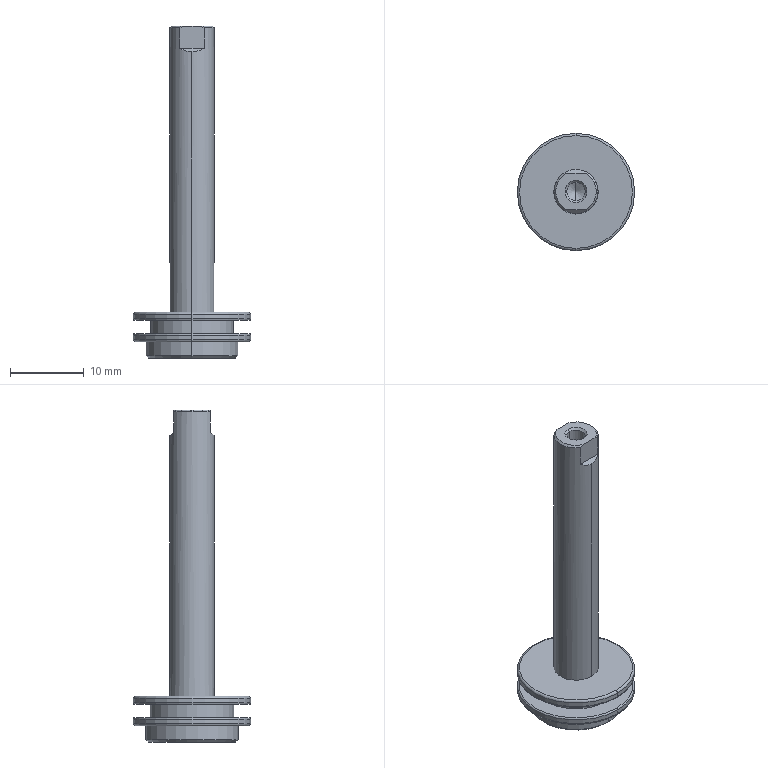Component | SolidWorks | SDA_16x25_0-1_SDA_16x2525_r-1 | 1 solid | 38 faces | box 15.9 x 15.9 x 45 mm | volume 1937 mm3 | cylinder 12 | plane 10 | cone 8 | torus 8 | commonest cylinder face diameters 15.9 x4 2.459 x2 12.5 x2 11.3 x2 6 x2
STEP:
#1=COLOUR_RGB('',0.7922,0.8196,0.9333);
#2=FILL_AREA_STYLE_COLOUR('',#1);
#3=FILL_AREA_STYLE('',(#2));
#4=SURFACE_STYLE_FILL_AREA(#3);
#5=SURFACE_SIDE_STYLE('',(#4));
#6=SURFACE_STYLE_USAGE(.BOTH.,#5);
#7=PRESENTATION_STYLE_ASSIGNMENT((#6));
#8=CARTESIAN_POINT('',(-0.2723,0.7951,0.8728));
#9=VERTEX_POINT('',#8);
#10=CARTESIAN_POINT('',(-0.2723,0.8435,0.9007));
#11=VERTEX_POINT('',#10);
#12=CARTESIAN_POINT('',(-0.2723,0.7951,0.8728));
#13=DIRECTION('',(0.,0.866,0.5));
#14=VECTOR('',#13,39.37);
#15=LINE('',#12,#14);
#16=EDGE_CURVE('',#9,#11,#15,.T.);
#17=ORIENTED_EDGE('',*,*,#16,.F.);
#18=CARTESIAN_POINT('',(-0.2723,0.7467,0.9007));
#19=VERTEX_POINT('',#18);
#20=CARTESIAN_POINT('',(-0.2723,0.7951,0.8728));
#21=DIRECTION('',(-0.,-0.866,0.5));
#22=VECTOR('',#21,39.37);
#23=LINE('',#20,#22);
#24=EDGE_CURVE('',#9,#19,#23,.T.);
#25=ORIENTED_EDGE('',*,*,#24,.T.);
#26=CARTESIAN_POINT('',(-0.2723,0.7951,0.9007));
#27=DIRECTION('',(-0.,0.,1.));
#28=DIRECTION('',(0.,1.,0.));
#29=AXIS2_PLACEMENT_3D('',#26,#27,#28);
#30=CIRCLE('',#29,0.04841);
#31=EDGE_CURVE('',#19,#11,#30,.T.);
#32=ORIENTED_EDGE('',*,*,#31,.T.);
#33=EDGE_LOOP('',(#17,#25,#32));
#34=FACE_OUTER_BOUND('',#33,.T.);
#35=CARTESIAN_POINT('',(-0.2723,0.7951,40.243));
#36=DIRECTION('',(-0.,0.,1.));
#37=DIRECTION('',(0.,1.,0.));
#38=AXIS2_PLACEMENT_3D('',#35,#36,#37);
#39=CONICAL_SURFACE('',#38,68.191,1.047);
#40=ADVANCED_FACE('',(#34),#39,.F.);
#41=ORIENTED_EDGE('',*,*,#31,.F.);
#42=CARTESIAN_POINT('',(-0.2723,0.7467,1.174));
#43=VERTEX_POINT('',#42);
#44=CARTESIAN_POINT('',(-0.2723,0.7467,0.8728));
#45=DIRECTION('',(-0.,0.,1.));
#46=VECTOR('',#45,39.37);
#47=LINE('',#44,#46);
#48=EDGE_CURVE('',#19,#43,#47,.T.);
#49=ORIENTED_EDGE('',*,*,#48,.T.);
#50=CARTESIAN_POINT('',(-0.2723,0.8435,1.174));
#51=VERTEX_POINT('',#50);
#52=CARTESIAN_POINT('',(-0.2723,0.7951,1.174));
#53=DIRECTION('',(-0.,0.,1.));
#54=DIRECTION('',(0.,1.,0.));
#55=AXIS2_PLACEMENT_3D('',#52,#53,#54);
#56=CIRCLE('',#55,0.04841);
#57=EDGE_CURVE('',#43,#51,#56,.T.);
#58=ORIENTED_EDGE('',*,*,#57,.T.);
#59=CARTESIAN_POINT('',(-0.2723,0.8435,0.8728));
#60=DIRECTION('',(-0.,0.,1.));
#61=VECTOR('',#60,39.37);
#62=LINE('',#59,#61);
#63=EDGE_CURVE('',#11,#51,#62,.T.);
#64=ORIENTED_EDGE('',*,*,#63,.F.);
#65=EDGE_LOOP('',(#41,#49,#58,#64));
#66=FACE_OUTER_BOUND('',#65,.T.);
#67=CARTESIAN_POINT('',(-0.2723,0.7951,0.8728));
#68=DIRECTION('',(-0.,0.,1.));
#69=DIRECTION('',(0.,1.,0.));
#70=AXIS2_PLACEMENT_3D('',#67,#68,#69);
#71=CYLINDRICAL_SURFACE('',#70,0.04841);
#72=ADVANCED_FACE('',(#66),#71,.F.);
#73=ORIENTED_EDGE('',*,*,#57,.F.);
#74=CARTESIAN_POINT('',(-0.2723,0.736,1.184));
#75=VERTEX_POINT('',#74);
#76=CARTESIAN_POINT('',(-0.2723,0.7467,1.174));
#77=DIRECTION('',(-0.,-0.7071,0.7071));
#78=VECTOR('',#77,39.37);
#79=LINE('',#76,#78);
#80=EDGE_CURVE('',#43,#75,#79,.T.);
#81=ORIENTED_EDGE('',*,*,#80,.T.);
#82=CARTESIAN_POINT('',(-0.2723,0.8541,1.184));
#83=VERTEX_POINT('',#82);
#84=CARTESIAN_POINT('',(-0.2723,0.7951,1.184));
#85=DIRECTION('',(-0.,0.,1.));
#86=DIRECTION('',(0.,1.,0.));
#87=AXIS2_PLACEMENT_3D('',#84,#85,#86);
#88=CIRCLE('',#87,0.05906);
#89=EDGE_CURVE('',#75,#83,#88,.T.);
#90=ORIENTED_EDGE('',*,*,#89,.T.);
#91=CARTESIAN_POINT('',(-0.2723,0.8435,1.174));
#92=DIRECTION('',(0.,0.7071,0.7071));
#93=VECTOR('',#92,39.37);
#94=LINE('',#91,#93);
#95=EDGE_CURVE('',#51,#83,#94,.T.);
#96=ORIENTED_EDGE('',*,*,#95,.F.);
#97=EDGE_LOOP('',(#73,#81,#90,#96));
#98=FACE_OUTER_BOUND('',#97,.T.);
#99=CARTESIAN_POINT('',(-0.2723,0.7951,1.174));
#100=DIRECTION('',(-0.,0.,1.));
#101=DIRECTION('',(0.,1.,0.));
#102=AXIS2_PLACEMENT_3D('',#99,#100,#101);
#103=CONICAL_SURFACE('',#102,0.04841,0.7854);
#104=ADVANCED_FACE('',(#98),#103,.F.);
#105=CARTESIAN_POINT('',(-0.2723,1.029,-0.5874));
#106=VERTEX_POINT('',#105);
#107=CARTESIAN_POINT('',(-0.2723,0.5608,-0.5874));
#108=VERTEX_POINT('',#107);
#109=CARTESIAN_POINT('',(-0.2723,0.7951,-0.5874));
#110=DIRECTION('',(-0.,0.,1.));
#111=DIRECTION('',(0.,1.,0.));
#112=AXIS2_PLACEMENT_3D('',#109,#110,#111);
#113=CIRCLE('',#112,0.2343);
#114=EDGE_CURVE('',#106,#108,#113,.T.);
#115=ORIENTED_EDGE('',*,*,#114,.T.);
#116=CARTESIAN_POINT('',(-0.2723,0.549,-0.5756));
#117=VERTEX_POINT('',#116);
#118=CARTESIAN_POINT('',(-0.2723,0.5608,-0.5874));
#119=DIRECTION('',(-0.,-0.7071,0.7071));
#120=VECTOR('',#119,39.37);
#121=LINE('',#118,#120);
#122=EDGE_CURVE('',#108,#117,#121,.T.);
#123=ORIENTED_EDGE('',*,*,#122,.T.);
#124=CARTESIAN_POINT('',(-0.2723,1.041,-0.5756));
#125=VERTEX_POINT('',#124);
#126=CARTESIAN_POINT('',(-0.2723,0.7951,-0.5756));
#127=DIRECTION('',(-0.,0.,1.));
#128=DIRECTION('',(0.,1.,0.));
#129=AXIS2_PLACEMENT_3D('',#126,#127,#128);
#130=CIRCLE('',#129,0.2461);
#131=EDGE_CURVE('',#125,#117,#130,.T.);
#132=ORIENTED_EDGE('',*,*,#131,.F.);
#133=CARTESIAN_POINT('',(-0.2723,1.029,-0.5874));
#134=DIRECTION('',(0.,0.7071,0.7071));
#135=VECTOR('',#134,39.37);
#136=LINE('',#133,#135);
#137=EDGE_CURVE('',#106,#125,#136,.T.);
#138=ORIENTED_EDGE('',*,*,#137,.F.);
#139=EDGE_LOOP('',(#115,#123,#132,#138));
#140=FACE_OUTER_BOUND('',#139,.T.);
#141=CARTESIAN_POINT('',(-0.2723,0.7951,-0.5874));
#142=DIRECTION('',(-0.,0.,1.));
#143=DIRECTION('',(0.,1.,0.));
#144=AXIS2_PLACEMENT_3D('',#141,#142,#143);
#145=CONICAL_SURFACE('',#144,0.2343,0.7854);
#146=ADVANCED_FACE('',(#140),#145,.T.);
#147=ORIENTED_EDGE('',*,*,#131,.T.);
#148=CARTESIAN_POINT('',(-0.2723,0.549,-0.5008));
#149=VERTEX_POINT('',#148);
#150=CARTESIAN_POINT('',(-0.2723,0.549,-0.5874));
#151=DIRECTION('',(-0.,0.,1.));
#152=VECTOR('',#151,39.37);
#153=LINE('',#150,#152);
#154=EDGE_CURVE('',#117,#149,#153,.T.);
#155=ORIENTED_EDGE('',*,*,#154,.T.);
#156=CARTESIAN_POINT('',(-0.2723,1.041,-0.5008));
#157=VERTEX_POINT('',#156);
#158=CARTESIAN_POINT('',(-0.2723,0.7951,-0.5008));
#159=DIRECTION('',(-0.,0.,1.));
#160=DIRECTION('',(0.,1.,0.));
#161=AXIS2_PLACEMENT_3D('',#158,#159,#160);
#162=CIRCLE('',#161,0.2461);
#163=EDGE_CURVE('',#157,#149,#162,.T.);
#164=ORIENTED_EDGE('',*,*,#163,.F.);
#165=CARTESIAN_POINT('',(-0.2723,1.041,-0.5874));
#166=DIRECTION('',(-0.,0.,1.));
#167=VECTOR('',#166,39.37);
#168=LINE('',#165,#167);
#169=EDGE_CURVE('',#125,#157,#168,.T.);
#170=ORIENTED_EDGE('',*,*,#169,.F.);
#171=EDGE_LOOP('',(#147,#155,#164,#170));
#172=FACE_OUTER_BOUND('',#171,.T.);
#173=CARTESIAN_POINT('',(-0.2723,0.7951,-0.5874));
#174=DIRECTION('',(-0.,0.,1.));
#175=DIRECTION('',(0.,1.,0.));
#176=AXIS2_PLACEMENT_3D('',#173,#174,#175);
#177=CYLINDRICAL_SURFACE('',#176,0.2461);
#178=ADVANCED_FACE('',(#172),#177,.T.);
#179=CARTESIAN_POINT('',(-0.2723,1.096,-0.5008));
#180=VERTEX_POINT('',#179);
#181=CARTESIAN_POINT('',(-0.2723,0.4939,-0.5008));
#182=VERTEX_POINT('',#181);
#183=CARTESIAN_POINT('',(-0.2723,0.7951,-0.5008));
#184=DIRECTION('',(-0.,0.,1.));
#185=DIRECTION('',(0.,1.,0.));
#186=AXIS2_PLACEMENT_3D('',#183,#184,#185);
#187=CIRCLE('',#186,0.3012);
#188=EDGE_CURVE('',#180,#182,#187,.T.);
#189=ORIENTED_EDGE('',*,*,#188,.T.);
#190=CARTESIAN_POINT('',(-0.2723,0.4821,-0.489));
#191=VERTEX_POINT('',#190);
#192=CARTESIAN_POINT('',(-0.2723,0.4939,-0.489));
#193=DIRECTION('',(-1.,0.,-0.));
#194=DIRECTION('',(-0.,-1.,0.));
#195=AXIS2_PLACEMENT_3D('',#192,#193,#194);
#196=CIRCLE('',#195,0.01181);
#197=EDGE_CURVE('',#182,#191,#196,.T.);
#198=ORIENTED_EDGE('',*,*,#197,.T.);
#199=CARTESIAN_POINT('',(-0.2723,1.108,-0.489));
#200=VERTEX_POINT('',#199);
#201=CARTESIAN_POINT('',(-0.2723,0.7951,-0.489));
#202=DIRECTION('',(-0.,0.,1.));
#203=DIRECTION('',(0.,1.,0.));
#204=AXIS2_PLACEMENT_3D('',#201,#202,#203);
#205=CIRCLE('',#204,0.313);
#206=EDGE_CURVE('',#200,#191,#205,.T.);
#207=ORIENTED_EDGE('',*,*,#206,.F.);
#208=CARTESIAN_POINT('',(-0.2723,1.096,-0.489));
#209=DIRECTION('',(1.,-0.,0.));
#210=DIRECTION('',(0.,1.,0.));
#211=AXIS2_PLACEMENT_3D('',#208,#209,#210);
#212=CIRCLE('',#211,0.01181);
#213=EDGE_CURVE('',#180,#200,#212,.T.);
#214=ORIENTED_EDGE('',*,*,#213,.F.);
#215=EDGE_LOOP('',(#189,#198,#207,#214));
#216=FACE_OUTER_BOUND('',#215,.T.);
#217=CARTESIAN_POINT('',(-0.2723,0.7951,-0.489));
#218=DIRECTION('',(-0.,0.,1.));
#219=DIRECTION('',(0.,1.,-0.));
#220=AXIS2_PLACEMENT_3D('',#217,#218,#219);
#221=TOROIDAL_SURFACE('',#220,0.3012,0.01181);
#222=ADVANCED_FACE('',(#216),#221,.T.);
#223=ORIENTED_EDGE('',*,*,#206,.T.);
#224=CARTESIAN_POINT('',(-0.2723,0.4821,-0.4654));
#225=VERTEX_POINT('',#224);
#226=CARTESIAN_POINT('',(-0.2723,0.4821,-0.5874));
#227=DIRECTION('',(-0.,0.,1.));
#228=VECTOR('',#227,39.37);
#229=LINE('',#226,#228);
#230=EDGE_CURVE('',#191,#225,#229,.T.);
#231=ORIENTED_EDGE('',*,*,#230,.T.);
#232=CARTESIAN_POINT('',(-0.2723,1.108,-0.4654));
#233=VERTEX_POINT('',#232);
#234=CARTESIAN_POINT('',(-0.2723,0.7951,-0.4654));
#235=DIRECTION('',(-0.,0.,1.));
#236=DIRECTION('',(0.,1.,0.));
#237=AXIS2_PLACEMENT_3D('',#234,#235,#236);
#238=CIRCLE('',#237,0.313);
#239=EDGE_CURVE('',#233,#225,#238,.T.);
#240=ORIENTED_EDGE('',*,*,#239,.F.);
#241=CARTESIAN_POINT('',(-0.2723,1.108,-0.5874));
#242=DIRECTION('',(-0.,0.,1.));
#243=VECTOR('',#242,39.37);
#244=LINE('',#241,#243);
#245=EDGE_CURVE('',#200,#233,#244,.T.);
#246=ORIENTED_EDGE('',*,*,#245,.F.);
#247=EDGE_LOOP('',(#223,#231,#240,#246));
#248=FACE_OUTER_BOUND('',#247,.T.);
#249=CARTESIAN_POINT('',(-0.2723,0.7951,-0.5874));
#250=DIRECTION('',(-0.,0.,1.));
#251=DIRECTION('',(0.,1.,0.));
#252=AXIS2_PLACEMENT_3D('',#249,#250,#251);
#253=CYLINDRICAL_SURFACE('',#252,0.313);
#254=ADVANCED_FACE('',(#248),#253,.T.);
#255=ORIENTED_EDGE('',*,*,#239,.T.);
#256=CARTESIAN_POINT('',(-0.2723,0.49,-0.4575));
#257=VERTEX_POINT('',#256);
#258=CARTESIAN_POINT('',(-0.2723,0.49,-0.4654));
#259=DIRECTION('',(-1.,0.,-0.));
#260=DIRECTION('',(-0.,-1.,0.));
#261=AXIS2_PLACEMENT_3D('',#258,#259,#260);
#262=CIRCLE('',#261,0.007874);
#263=EDGE_CURVE('',#225,#257,#262,.T.);
#264=ORIENTED_EDGE('',*,*,#263,.T.);
#265=CARTESIAN_POINT('',(-0.2723,1.1,-0.4575));
#266=VERTEX_POINT('',#265);
#267=CARTESIAN_POINT('',(-0.2723,0.7951,-0.4575));
#268=DIRECTION('',(-0.,0.,1.));
#269=DIRECTION('',(0.,1.,0.));
#270=AXIS2_PLACEMENT_3D('',#267,#268,#269);
#271=CIRCLE('',#270,0.3051);
#272=EDGE_CURVE('',#266,#257,#271,.T.);
#273=ORIENTED_EDGE('',*,*,#272,.F.);
#274=CARTESIAN_POINT('',(-0.2723,1.1,-0.4654));
#275=DIRECTION('',(1.,-0.,0.));
#276=DIRECTION('',(0.,1.,0.));
#277=AXIS2_PLACEMENT_3D('',#274,#275,#276);
#278=CIRCLE('',#277,0.007874);
#279=EDGE_CURVE('',#233,#266,#278,.T.);
#280=ORIENTED_EDGE('',*,*,#279,.F.);
#281=EDGE_LOOP('',(#255,#264,#273,#280));
#282=FACE_OUTER_BOUND('',#281,.T.);
#283=CARTESIAN_POINT('',(-0.2723,0.7951,-0.4654));
#284=DIRECTION('',(-0.,0.,1.));
#285=DIRECTION('',(0.,1.,-0.));
#286=AXIS2_PLACEMENT_3D('',#283,#284,#285);
#287=TOROIDAL_SURFACE('',#286,0.3051,0.007874);
#288=ADVANCED_FACE('',(#282),#287,.T.);
#289=CARTESIAN_POINT('',(-0.2723,1.018,-0.4575));
#290=VERTEX_POINT('',#289);
#291=CARTESIAN_POINT('',(-0.2723,0.5726,-0.4575));
#292=VERTEX_POINT('',#291);
#293=CARTESIAN_POINT('',(-0.2723,0.7951,-0.4575));
#294=DIRECTION('',(-0.,0.,1.));
#295=DIRECTION('',(0.,1.,0.));
#296=AXIS2_PLACEMENT_3D('',#293,#294,#295);
#297=CIRCLE('',#296,0.2224);
#298=EDGE_CURVE('',#290,#292,#297,.T.);
#299=ORIENTED_EDGE('',*,*,#298,.T.);
#300=CARTESIAN_POINT('',(-0.2723,0.5726,-0.3867));
#301=VERTEX_POINT('',#300);
#302=CARTESIAN_POINT('',(-0.2723,0.5726,-0.5874));
#303=DIRECTION('',(-0.,0.,1.));
#304=VECTOR('',#303,39.37);
#305=LINE('',#302,#304);
#306=EDGE_CURVE('',#292,#301,#305,.T.);
#307=ORIENTED_EDGE('',*,*,#306,.T.);
#308=CARTESIAN_POINT('',(-0.2723,1.018,-0.3867));
#309=VERTEX_POINT('',#308);
#310=CARTESIAN_POINT('',(-0.2723,0.7951,-0.3867));
#311=DIRECTION('',(-0.,0.,1.));
#312=DIRECTION('',(0.,1.,0.));
#313=AXIS2_PLACEMENT_3D('',#310,#311,#312);
#314=CIRCLE('',#313,0.2224);
#315=EDGE_CURVE('',#309,#301,#314,.T.);
#316=ORIENTED_EDGE('',*,*,#315,.F.);
#317=CARTESIAN_POINT('',(-0.2723,1.018,-0.5874));
#318=DIRECTION('',(-0.,0.,1.));
#319=VECTOR('',#318,39.37);
#320=LINE('',#317,#319);
#321=EDGE_CURVE('',#290,#309,#320,.T.);
#322=ORIENTED_EDGE('',*,*,#321,.F.);
#323=EDGE_LOOP('',(#299,#307,#316,#322));
#324=FACE_OUTER_BOUND('',#323,.T.);
#325=CARTESIAN_POINT('',(-0.2723,0.7951,-0.5874));
#326=DIRECTION('',(-0.,0.,1.));
#327=DIRECTION('',(0.,1.,0.));
#328=AXIS2_PLACEMENT_3D('',#325,#326,#327);
#329=CYLINDRICAL_SURFACE('',#328,0.2224);
#330=ADVANCED_FACE('',(#324),#329,.T.);
#331=CARTESIAN_POINT('',(-0.2723,1.1,-0.3867));
#332=VERTEX_POINT('',#331);
#333=CARTESIAN_POINT('',(-0.2723,0.49,-0.3867));
#334=VERTEX_POINT('',#333);
#335=CARTESIAN_POINT('',(-0.2723,0.7951,-0.3867));
#336=DIRECTION('',(-0.,0.,1.));
#337=DIRECTION('',(0.,1.,0.));
#338=AXIS2_PLACEMENT_3D('',#335,#336,#337);
#339=CIRCLE('',#338,0.3051);
#340=EDGE_CURVE('',#332,#334,#339,.T.);
#341=ORIENTED_EDGE('',*,*,#340,.T.);
#342=CARTESIAN_POINT('',(-0.2723,0.4821,-0.3788));
#343=VERTEX_POINT('',#342);
#344=CARTESIAN_POINT('',(-0.2723,0.49,-0.3788));
#345=DIRECTION('',(-1.,0.,-0.));
#346=DIRECTION('',(-0.,-1.,0.));
#347=AXIS2_PLACEMENT_3D('',#344,#345,#346);
#348=CIRCLE('',#347,0.007874);
#349=EDGE_CURVE('',#334,#343,#348,.T.);
#350=ORIENTED_EDGE('',*,*,#349,.T.);
#351=CARTESIAN_POINT('',(-0.2723,1.108,-0.3788));
#352=VERTEX_POINT('',#351);
#353=CARTESIAN_POINT('',(-0.2723,0.7951,-0.3788));
#354=DIRECTION('',(-0.,0.,1.));
#355=DIRECTION('',(0.,1.,0.));
#356=AXIS2_PLACEMENT_3D('',#353,#354,#355);
#357=CIRCLE('',#356,0.313);
#358=EDGE_CURVE('',#352,#343,#357,.T.);
#359=ORIENTED_EDGE('',*,*,#358,.F.);
#360=CARTESIAN_POINT('',(-0.2723,1.1,-0.3788));
#361=DIRECTION('',(1.,-0.,0.));
#362=DIRECTION('',(0.,1.,0.));
#363=AXIS2_PLACEMENT_3D('',#360,#361,#362);
#364=CIRCLE('',#363,0.007874);
#365=EDGE_CURVE('',#332,#352,#364,.T.);
#366=ORIENTED_EDGE('',*,*,#365,.F.);
#367=EDGE_LOOP('',(#341,#350,#359,#366));
#368=FACE_OUTER_BOUND('',#367,.T.);
#369=CARTESIAN_POINT('',(-0.2723,0.7951,-0.3788));
#370=DIRECTION('',(-0.,0.,1.));
#371=DIRECTION('',(0.,1.,-0.));
#372=AXIS2_PLACEMENT_3D('',#369,#370,#371);
#373=TOROIDAL_SURFACE('',#372,0.3051,0.007874);
#374=ADVANCED_FACE('',(#368),#373,.T.);
#375=ORIENTED_EDGE('',*,*,#358,.T.);
#376=CARTESIAN_POINT('',(-0.2723,0.4821,-0.3552));
#377=VERTEX_POINT('',#376);
#378=CARTESIAN_POINT('',(-0.2723,0.4821,-0.5874));
#379=DIRECTION('',(-0.,0.,1.));
#380=VECTOR('',#379,39.37);
#381=LINE('',#378,#380);
#382=EDGE_CURVE('',#343,#377,#381,.T.);
#383=ORIENTED_EDGE('',*,*,#382,.T.);
#384=CARTESIAN_POINT('',(-0.2723,1.108,-0.3552));
#385=VERTEX_POINT('',#384);
#386=CARTESIAN_POINT('',(-0.2723,0.7951,-0.3552));
#387=DIRECTION('',(-0.,0.,1.));
#388=DIRECTION('',(0.,1.,0.));
#389=AXIS2_PLACEMENT_3D('',#386,#387,#388);
#390=CIRCLE('',#389,0.313);
#391=EDGE_CURVE('',#385,#377,#390,.T.);
#392=ORIENTED_EDGE('',*,*,#391,.F.);
#393=CARTESIAN_POINT('',(-0.2723,1.108,-0.5874));
#394=DIRECTION('',(-0.,0.,1.));
#395=VECTOR('',#394,39.37);
#396=LINE('',#393,#395);
#397=EDGE_CURVE('',#352,#385,#396,.T.);
#398=ORIENTED_EDGE('',*,*,#397,.F.);
#399=EDGE_LOOP('',(#375,#383,#392,#398));
#400=FACE_OUTER_BOUND('',#399,.T.);
#401=CARTESIAN_POINT('',(-0.2723,0.7951,-0.5874));
#402=DIRECTION('',(-0.,0.,1.));
#403=DIRECTION('',(0.,1.,0.));
#404=AXIS2_PLACEMENT_3D('',#401,#402,#403);
#405=CYLINDRICAL_SURFACE('',#404,0.313);
#406=ADVANCED_FACE('',(#400),#405,.T.);
#407=ORIENTED_EDGE('',*,*,#391,.T.);
#408=CARTESIAN_POINT('',(-0.2723,0.4939,-0.3433));
#409=VERTEX_POINT('',#408);
#410=CARTESIAN_POINT('',(-0.2723,0.4939,-0.3552));
#411=DIRECTION('',(-1.,0.,-0.));
#412=DIRECTION('',(-0.,-1.,0.));
#413=AXIS2_PLACEMENT_3D('',#410,#411,#412);
#414=CIRCLE('',#413,0.01181);
#415=EDGE_CURVE('',#377,#409,#414,.T.);
#416=ORIENTED_EDGE('',*,*,#415,.T.);
#417=CARTESIAN_POINT('',(-0.2723,1.096,-0.3433));
#418=VERTEX_POINT('',#417);
#419=CARTESIAN_POINT('',(-0.2723,0.7951,-0.3433));
#420=DIRECTION('',(-0.,0.,1.));
#421=DIRECTION('',(0.,1.,0.));
#422=AXIS2_PLACEMENT_3D('',#419,#420,#421);
#423=CIRCLE('',#422,0.3012);
#424=EDGE_CURVE('',#418,#409,#423,.T.);
#425=ORIENTED_EDGE('',*,*,#424,.F.);
#426=CARTESIAN_POINT('',(-0.2723,1.096,-0.3552));
#427=DIRECTION('',(1.,-0.,0.));
#428=DIRECTION('',(0.,1.,0.));
#429=AXIS2_PLACEMENT_3D('',#426,#427,#428);
#430=CIRCLE('',#429,0.01181);
#431=EDGE_CURVE('',#385,#418,#430,.T.);
#432=ORIENTED_EDGE('',*,*,#431,.F.);
#433=EDGE_LOOP('',(#407,#416,#425,#432));
#434=FACE_OUTER_BOUND('',#433,.T.);
#435=CARTESIAN_POINT('',(-0.2723,0.7951,-0.3552));
#436=DIRECTION('',(-0.,0.,1.));
#437=DIRECTION('',(0.,1.,-0.));
#438=AXIS2_PLACEMENT_3D('',#435,#436,#437);
#439=TOROIDAL_SURFACE('',#438,0.3012,0.01181);
#440=ADVANCED_FACE('',(#434),#439,.T.);
#441=CARTESIAN_POINT('',(-0.2723,0.9132,-0.3433));
#442=VERTEX_POINT('',#441);
#443=CARTESIAN_POINT('',(-0.2723,0.677,-0.3433));
#444=VERTEX_POINT('',#443);
#445=CARTESIAN_POINT('',(-0.2723,0.7951,-0.3433));
#446=DIRECTION('',(-0.,0.,1.));
#447=DIRECTION('',(0.,1.,0.));
#448=AXIS2_PLACEMENT_3D('',#445,#446,#447);
#449=CIRCLE('',#448,0.1181);
#450=EDGE_CURVE('',#442,#444,#449,.T.);
#451=ORIENTED_EDGE('',*,*,#450,.T.);
#452=CARTESIAN_POINT('',(-0.2723,0.677,1.046));
#453=VERTEX_POINT('',#452);
#454=CARTESIAN_POINT('',(-0.2723,0.677,0.9677));
#455=DIRECTION('',(-0.,0.,1.));
#456=VECTOR('',#455,39.37);
#457=LINE('',#454,#456);
#458=EDGE_CURVE('',#444,#453,#457,.T.);
#459=ORIENTED_EDGE('',*,*,#458,.T.);
#460=CARTESIAN_POINT('',(-0.3376,0.6967,1.066));
#461=VERTEX_POINT('',#460);
#462=CARTESIAN_POINT('',(-0.2723,0.677,1.046));
#463=CARTESIAN_POINT('',(-0.2957,0.677,1.046));
#464=CARTESIAN_POINT('',(-0.3181,0.6837,1.053));
#465=CARTESIAN_POINT('',(-0.3376,0.6967,1.066));
#466=(BOUNDED_CURVE()B_SPLINE_CURVE(3,(#462,#463,#464,#465),.UNSPECIFIED.,.F.,.F.)B_SPLINE_CURVE_WITH_KNOTS((4,4),(3.142,3.727),.UNSPECIFIED.)CURVE()GEOMETRIC_REPRESENTATION_ITEM()RATIONAL_B_SPLINE_CURVE((1.,0.9716,0.9716,1.))REPRESENTATION_ITEM(''));
#467=EDGE_CURVE('',#453,#461,#466,.T.);
#468=ORIENTED_EDGE('',*,*,#467,.T.);
#469=CARTESIAN_POINT('',(-0.3376,0.6967,1.174));
#470=VERTEX_POINT('',#469);
#471=CARTESIAN_POINT('',(-0.3376,0.6967,0.9677));
#472=DIRECTION('',(-0.,0.,1.));
#473=VECTOR('',#472,39.37);
#474=LINE('',#471,#473);
#475=EDGE_CURVE('',#461,#470,#474,.T.);
#476=ORIENTED_EDGE('',*,*,#475,.T.);
#477=CARTESIAN_POINT('',(-0.3376,0.8935,1.174));
#478=VERTEX_POINT('',#477);
#479=CARTESIAN_POINT('',(-0.2723,0.7951,1.174));
#480=DIRECTION('',(-0.,0.,1.));
#481=DIRECTION('',(0.,1.,0.));
#482=AXIS2_PLACEMENT_3D('',#479,#480,#481);
#483=CIRCLE('',#482,0.1181);
#484=EDGE_CURVE('',#478,#470,#483,.T.);
#485=ORIENTED_EDGE('',*,*,#484,.F.);
#486=CARTESIAN_POINT('',(-0.3376,0.8935,1.066));
#487=VERTEX_POINT('',#486);
#488=CARTESIAN_POINT('',(-0.3376,0.8935,0.9677));
#489=DIRECTION('',(0.,-0.,-1.));
#490=VECTOR('',#489,39.37);
#491=LINE('',#488,#490);
#492=EDGE_CURVE('',#478,#487,#491,.T.);
#493=ORIENTED_EDGE('',*,*,#492,.T.);
#494=CARTESIAN_POINT('',(-0.2723,0.9132,1.046));
#495=VERTEX_POINT('',#494);
#496=CARTESIAN_POINT('',(-0.3376,0.8935,1.066));
#497=CARTESIAN_POINT('',(-0.3181,0.9064,1.053));
#498=CARTESIAN_POINT('',(-0.2957,0.9132,1.046));
#499=CARTESIAN_POINT('',(-0.2723,0.9132,1.046));
#500=(BOUNDED_CURVE()B_SPLINE_CURVE(3,(#496,#497,#498,#499),.UNSPECIFIED.,.F.,.F.)B_SPLINE_CURVE_WITH_KNOTS((4,4),(2.556,3.142),.UNSPECIFIED.)CURVE()GEOMETRIC_REPRESENTATION_ITEM()RATIONAL_B_SPLINE_CURVE((1.,0.9716,0.9716,1.))REPRESENTATION_ITEM(''));
#501=EDGE_CURVE('',#487,#495,#500,.T.);
#502=ORIENTED_EDGE('',*,*,#501,.T.);
#503=CARTESIAN_POINT('',(-0.2723,0.9132,0.9677));
#504=DIRECTION('',(-0.,0.,1.));
#505=VECTOR('',#504,39.37);
#506=LINE('',#503,#505);
#507=EDGE_CURVE('',#442,#495,#506,.T.);
#508=ORIENTED_EDGE('',*,*,#507,.F.);
#509=EDGE_LOOP('',(#451,#459,#468,#476,#485,#493,#502,#508));
#510=FACE_OUTER_BOUND('',#509,.T.);
#511=CARTESIAN_POINT('',(-0.2723,0.7951,0.9677));
#512=DIRECTION('',(-0.,0.,1.));
#513=DIRECTION('',(0.,1.,0.));
#514=AXIS2_PLACEMENT_3D('',#511,#512,#513);
#515=CYLINDRICAL_SURFACE('',#514,0.1181);
#516=ADVANCED_FACE('',(#510),#515,.T.);
#517=CARTESIAN_POINT('',(-0.3174,0.8935,1.184));
#518=VERTEX_POINT('',#517);
#519=CARTESIAN_POINT('',(-0.3174,0.6967,1.184));
#520=VERTEX_POINT('',#519);
#521=CARTESIAN_POINT('',(-0.2723,0.7951,1.184));
#522=DIRECTION('',(-0.,0.,1.));
#523=DIRECTION('',(0.,1.,0.));
#524=AXIS2_PLACEMENT_3D('',#521,#522,#523);
#525=CIRCLE('',#524,0.1083);
#526=EDGE_CURVE('',#518,#520,#525,.T.);
#527=ORIENTED_EDGE('',*,*,#526,.T.);
#528=CARTESIAN_POINT('',(-0.2272,0.6967,1.184));
#529=VERTEX_POINT('',#528);
#530=CARTESIAN_POINT('',(-0.07542,0.6967,1.184));
#531=DIRECTION('',(-1.,0.,-0.));
#532=VECTOR('',#531,39.37);
#533=LINE('',#530,#532);
#534=EDGE_CURVE('',#529,#520,#533,.T.);
#535=ORIENTED_EDGE('',*,*,#534,.F.);
#536=CARTESIAN_POINT('',(-0.2272,0.8935,1.184));
#537=VERTEX_POINT('',#536);
#538=CARTESIAN_POINT('',(-0.2723,0.7951,1.184));
#539=DIRECTION('',(-0.,0.,1.));
#540=DIRECTION('',(0.,1.,0.));
#541=AXIS2_PLACEMENT_3D('',#538,#539,#540);
#542=CIRCLE('',#541,0.1083);
#543=EDGE_CURVE('',#529,#537,#542,.T.);
#544=ORIENTED_EDGE('',*,*,#543,.T.);
#545=CARTESIAN_POINT('',(-0.07542,0.8935,1.184));
#546=DIRECTION('',(-1.,0.,-0.));
#547=VECTOR('',#546,39.37);
#548=LINE('',#545,#547);
#549=EDGE_CURVE('',#537,#518,#548,.T.);
#550=ORIENTED_EDGE('',*,*,#549,.T.);
#551=EDGE_LOOP('',(#527,#535,#544,#550));
#552=FACE_OUTER_BOUND('',#551,.T.);
#553=CARTESIAN_POINT('',(-0.2723,0.7951,1.184));
#554=DIRECTION('',(-0.,0.,1.));
#555=DIRECTION('',(0.,1.,0.));
#556=AXIS2_PLACEMENT_3D('',#553,#554,#555);
#557=CIRCLE('',#556,0.05906);
#558=EDGE_CURVE('',#83,#75,#557,.T.);
#559=ORIENTED_EDGE('',*,*,#558,.F.);
#560=ORIENTED_EDGE('',*,*,#89,.F.);
#561=EDGE_LOOP('',(#559,#560));
#562=FACE_BOUND('',#561,.T.);
#563=CARTESIAN_POINT('',(-0.2723,0.7951,1.184));
#564=DIRECTION('',(0.,-0.,-1.));
#565=DIRECTION('',(-0.,-1.,0.));
#566=AXIS2_PLACEMENT_3D('',#563,#564,#565);
#567=PLANE('',#566);
#568=ADVANCED_FACE('',(#552,#562),#567,.F.);
#569=ORIENTED_EDGE('',*,*,#484,.T.);
#570=CARTESIAN_POINT('',(-0.3376,0.6967,1.174));
#571=CARTESIAN_POINT('',(-0.331,0.6967,1.178));
#572=CARTESIAN_POINT('',(-0.3243,0.6967,1.181));
#573=CARTESIAN_POINT('',(-0.3174,0.6967,1.184));
#574=B_SPLINE_CURVE_WITH_KNOTS('',3,(#570,#571,#572,#573),.UNSPECIFIED.,.F.,.F.,(4,4),(0.00574,0.006311),.UNSPECIFIED.);
#575=EDGE_CURVE('',#470,#520,#574,.T.);
#576=ORIENTED_EDGE('',*,*,#575,.T.);
#577=ORIENTED_EDGE('',*,*,#526,.F.);
#578=CARTESIAN_POINT('',(-0.3174,0.8935,1.184));
#579=CARTESIAN_POINT('',(-0.3243,0.8935,1.181));
#580=CARTESIAN_POINT('',(-0.331,0.8935,1.178));
#581=CARTESIAN_POINT('',(-0.3376,0.8935,1.174));
#582=B_SPLINE_CURVE_WITH_KNOTS('',3,(#578,#579,#580,#581),.UNSPECIFIED.,.F.,.F.,(4,4),(0.008672,0.009248),.UNSPECIFIED.);
#583=EDGE_CURVE('',#518,#478,#582,.T.);
#584=ORIENTED_EDGE('',*,*,#583,.T.);
#585=EDGE_LOOP('',(#569,#576,#577,#584));
#586=FACE_OUTER_BOUND('',#585,.T.);
#587=CARTESIAN_POINT('',(-0.2723,0.7951,1.174));
#588=DIRECTION('',(0.,-0.,-1.));
#589=DIRECTION('',(-0.,-1.,0.));
#590=AXIS2_PLACEMENT_3D('',#587,#588,#589);
#591=CONICAL_SURFACE('',#590,0.1181,0.7854);
#592=ADVANCED_FACE('',(#586),#591,.T.);
#593=ORIENTED_EDGE('',*,*,#543,.F.);
#594=CARTESIAN_POINT('',(-0.207,0.6967,1.174));
#595=VERTEX_POINT('',#594);
#596=CARTESIAN_POINT('',(-0.2272,0.6967,1.184));
#597=CARTESIAN_POINT('',(-0.2202,0.6967,1.181));
#598=CARTESIAN_POINT('',(-0.2135,0.6967,1.178));
#599=CARTESIAN_POINT('',(-0.207,0.6967,1.174));
#600=B_SPLINE_CURVE_WITH_KNOTS('',3,(#596,#597,#598,#599),.UNSPECIFIED.,.F.,.F.,(4,4),(0.008672,0.009248),.UNSPECIFIED.);
#601=EDGE_CURVE('',#529,#595,#600,.T.);
#602=ORIENTED_EDGE('',*,*,#601,.T.);
#603=CARTESIAN_POINT('',(-0.207,0.8935,1.174));
#604=VERTEX_POINT('',#603);
#605=CARTESIAN_POINT('',(-0.2723,0.7951,1.174));
#606=DIRECTION('',(-0.,0.,1.));
#607=DIRECTION('',(0.,1.,0.));
#608=AXIS2_PLACEMENT_3D('',#605,#606,#607);
#609=CIRCLE('',#608,0.1181);
#610=EDGE_CURVE('',#595,#604,#609,.T.);
#611=ORIENTED_EDGE('',*,*,#610,.T.);
#612=CARTESIAN_POINT('',(-0.207,0.8935,1.174));
#613=CARTESIAN_POINT('',(-0.2135,0.8935,1.178));
#614=CARTESIAN_POINT('',(-0.2202,0.8935,1.181));
#615=CARTESIAN_POINT('',(-0.2272,0.8935,1.184));
#616=B_SPLINE_CURVE_WITH_KNOTS('',3,(#612,#613,#614,#615),.UNSPECIFIED.,.F.,.F.,(4,4),(0.00574,0.006311),.UNSPECIFIED.);
#617=EDGE_CURVE('',#604,#537,#616,.T.);
#618=ORIENTED_EDGE('',*,*,#617,.T.);
#619=EDGE_LOOP('',(#593,#602,#611,#618));
#620=FACE_OUTER_BOUND('',#619,.T.);
#621=CARTESIAN_POINT('',(-0.2723,0.7951,1.174));
#622=DIRECTION('',(0.,-0.,-1.));
#623=DIRECTION('',(-0.,-1.,0.));
#624=AXIS2_PLACEMENT_3D('',#621,#622,#623);
#625=CONICAL_SURFACE('',#624,0.1181,0.7854);
#626=ADVANCED_FACE('',(#620),#625,.T.);
#627=ORIENTED_EDGE('',*,*,#458,.F.);
#628=CARTESIAN_POINT('',(-0.2723,0.7951,-0.3433));
#629=DIRECTION('',(-0.,0.,1.));
#630=DIRECTION('',(0.,1.,0.));
#631=AXIS2_PLACEMENT_3D('',#628,#629,#630);
#632=CIRCLE('',#631,0.1181);
#633=EDGE_CURVE('',#444,#442,#632,.T.);
#634=ORIENTED_EDGE('',*,*,#633,.T.);
#635=ORIENTED_EDGE('',*,*,#507,.T.);
#636=CARTESIAN_POINT('',(-0.207,0.8935,1.066));
#637=VERTEX_POINT('',#636);
#638=CARTESIAN_POINT('',(-0.2723,0.9132,1.046));
#639=CARTESIAN_POINT('',(-0.2489,0.9132,1.046));
#640=CARTESIAN_POINT('',(-0.2265,0.9064,1.053));
#641=CARTESIAN_POINT('',(-0.207,0.8935,1.066));
#642=(BOUNDED_CURVE()B_SPLINE_CURVE(3,(#638,#639,#640,#641),.UNSPECIFIED.,.F.,.F.)B_SPLINE_CURVE_WITH_KNOTS((4,4),(3.142,3.727),.UNSPECIFIED.)CURVE()GEOMETRIC_REPRESENTATION_ITEM()RATIONAL_B_SPLINE_CURVE((1.,0.9716,0.9716,1.))REPRESENTATION_ITEM(''));
#643=EDGE_CURVE('',#495,#637,#642,.T.);
#644=ORIENTED_EDGE('',*,*,#643,.T.);
#645=CARTESIAN_POINT('',(-0.207,0.8935,0.9677));
#646=DIRECTION('',(-0.,0.,1.));
#647=VECTOR('',#646,39.37);
#648=LINE('',#645,#647);
#649=EDGE_CURVE('',#637,#604,#648,.T.);
#650=ORIENTED_EDGE('',*,*,#649,.T.);
#651=ORIENTED_EDGE('',*,*,#610,.F.);
#652=CARTESIAN_POINT('',(-0.207,0.6967,1.066));
#653=VERTEX_POINT('',#652);
#654=CARTESIAN_POINT('',(-0.207,0.6967,0.9677));
#655=DIRECTION('',(0.,-0.,-1.));
#656=VECTOR('',#655,39.37);
#657=LINE('',#654,#656);
#658=EDGE_CURVE('',#595,#653,#657,.T.);
#659=ORIENTED_EDGE('',*,*,#658,.T.);
#660=CARTESIAN_POINT('',(-0.207,0.6967,1.066));
#661=CARTESIAN_POINT('',(-0.2265,0.6837,1.053));
#662=CARTESIAN_POINT('',(-0.2489,0.677,1.046));
#663=CARTESIAN_POINT('',(-0.2723,0.677,1.046));
#664=(BOUNDED_CURVE()B_SPLINE_CURVE(3,(#660,#661,#662,#663),.UNSPECIFIED.,.F.,.F.)B_SPLINE_CURVE_WITH_KNOTS((4,4),(2.556,3.142),.UNSPECIFIED.)CURVE()GEOMETRIC_REPRESENTATION_ITEM()RATIONAL_B_SPLINE_CURVE((1.,0.9716,0.9716,1.))REPRESENTATION_ITEM(''));
#665=EDGE_CURVE('',#653,#453,#664,.T.);
#666=ORIENTED_EDGE('',*,*,#665,.T.);
#667=EDGE_LOOP('',(#627,#634,#635,#644,#650,#651,#659,#666));
#668=FACE_OUTER_BOUND('',#667,.T.);
#669=CARTESIAN_POINT('',(-0.2723,0.7951,0.9677));
#670=DIRECTION('',(-0.,0.,1.));
#671=DIRECTION('',(0.,1.,0.));
#672=AXIS2_PLACEMENT_3D('',#669,#670,#671);
#673=CYLINDRICAL_SURFACE('',#672,0.1181);
#674=ADVANCED_FACE('',(#668),#673,.T.);
#675=ORIENTED_EDGE('',*,*,#450,.F.);
#676=ORIENTED_EDGE('',*,*,#633,.F.);
#677=EDGE_LOOP('',(#675,#676));
#678=FACE_BOUND('',#677,.T.);
#679=ORIENTED_EDGE('',*,*,#424,.T.);
#680=CARTESIAN_POINT('',(-0.2723,0.7951,-0.3433));
#681=DIRECTION('',(-0.,0.,1.));
#682=DIRECTION('',(0.,1.,0.));
#683=AXIS2_PLACEMENT_3D('',#680,#681,#682);
#684=CIRCLE('',#683,0.3012);
#685=EDGE_CURVE('',#409,#418,#684,.T.);
#686=ORIENTED_EDGE('',*,*,#685,.T.);
#687=EDGE_LOOP('',(#679,#686));
#688=FACE_OUTER_BOUND('',#687,.T.);
#689=CARTESIAN_POINT('',(-0.3904,0.7951,-0.3433));
#690=DIRECTION('',(0.,-0.,-1.));
#691=DIRECTION('',(-0.,-1.,0.));
#692=AXIS2_PLACEMENT_3D('',#689,#690,#691);
#693=PLANE('',#692);
#694=ADVANCED_FACE('',(#678,#688),#693,.F.);
#695=ORIENTED_EDGE('',*,*,#415,.F.);
#696=CARTESIAN_POINT('',(-0.2723,0.7951,-0.3552));
#697=DIRECTION('',(-0.,0.,1.));
#698=DIRECTION('',(0.,1.,0.));
#699=AXIS2_PLACEMENT_3D('',#696,#697,#698);
#700=CIRCLE('',#699,0.313);
#701=EDGE_CURVE('',#377,#385,#700,.T.);
#702=ORIENTED_EDGE('',*,*,#701,.T.);
#703=ORIENTED_EDGE('',*,*,#431,.T.);
#704=ORIENTED_EDGE('',*,*,#685,.F.);
#705=EDGE_LOOP('',(#695,#702,#703,#704));
#706=FACE_OUTER_BOUND('',#705,.T.);
#707=CARTESIAN_POINT('',(-0.2723,0.7951,-0.3552));
#708=DIRECTION('',(-0.,0.,1.));
#709=DIRECTION('',(0.,1.,-0.));
#710=AXIS2_PLACEMENT_3D('',#707,#708,#709);
#711=TOROIDAL_SURFACE('',#710,0.3012,0.01181);
#712=ADVANCED_FACE('',(#706),#711,.T.);
#713=ORIENTED_EDGE('',*,*,#382,.F.);
#714=CARTESIAN_POINT('',(-0.2723,0.7951,-0.3788));
#715=DIRECTION('',(-0.,0.,1.));
#716=DIRECTION('',(0.,1.,0.));
#717=AXIS2_PLACEMENT_3D('',#714,#715,#716);
#718=CIRCLE('',#717,0.313);
#719=EDGE_CURVE('',#343,#352,#718,.T.);
#720=ORIENTED_EDGE('',*,*,#719,.T.);
#721=ORIENTED_EDGE('',*,*,#397,.T.);
#722=ORIENTED_EDGE('',*,*,#701,.F.);
#723=EDGE_LOOP('',(#713,#720,#721,#722));
#724=FACE_OUTER_BOUND('',#723,.T.);
#725=CARTESIAN_POINT('',(-0.2723,0.7951,-0.5874));
#726=DIRECTION('',(-0.,0.,1.));
#727=DIRECTION('',(0.,1.,0.));
#728=AXIS2_PLACEMENT_3D('',#725,#726,#727);
#729=CYLINDRICAL_SURFACE('',#728,0.313);
#730=ADVANCED_FACE('',(#724),#729,.T.);
#731=ORIENTED_EDGE('',*,*,#349,.F.);
#732=CARTESIAN_POINT('',(-0.2723,0.7951,-0.3867));
#733=DIRECTION('',(-0.,0.,1.));
#734=DIRECTION('',(0.,1.,0.));
#735=AXIS2_PLACEMENT_3D('',#732,#733,#734);
#736=CIRCLE('',#735,0.3051);
#737=EDGE_CURVE('',#334,#332,#736,.T.);
#738=ORIENTED_EDGE('',*,*,#737,.T.);
#739=ORIENTED_EDGE('',*,*,#365,.T.);
#740=ORIENTED_EDGE('',*,*,#719,.F.);
#741=EDGE_LOOP('',(#731,#738,#739,#740));
#742=FACE_OUTER_BOUND('',#741,.T.);
#743=CARTESIAN_POINT('',(-0.2723,0.7951,-0.3788));
#744=DIRECTION('',(-0.,0.,1.));
#745=DIRECTION('',(0.,1.,-0.));
#746=AXIS2_PLACEMENT_3D('',#743,#744,#745);
#747=TOROIDAL_SURFACE('',#746,0.3051,0.007874);
#748=ADVANCED_FACE('',(#742),#747,.T.);
#749=ORIENTED_EDGE('',*,*,#340,.F.);
#750=ORIENTED_EDGE('',*,*,#737,.F.);
#751=EDGE_LOOP('',(#749,#750));
#752=FACE_OUTER_BOUND('',#751,.T.);
#753=ORIENTED_EDGE('',*,*,#315,.T.);
#754=CARTESIAN_POINT('',(-0.2723,0.7951,-0.3867));
#755=DIRECTION('',(-0.,0.,1.));
#756=DIRECTION('',(0.,1.,0.));
#757=AXIS2_PLACEMENT_3D('',#754,#755,#756);
#758=CIRCLE('',#757,0.2224);
#759=EDGE_CURVE('',#301,#309,#758,.T.);
#760=ORIENTED_EDGE('',*,*,#759,.T.);
#761=EDGE_LOOP('',(#753,#760));
#762=FACE_BOUND('',#761,.T.);
#763=CARTESIAN_POINT('',(-0.5774,0.7951,-0.3867));
#764=DIRECTION('',(-0.,0.,1.));
#765=DIRECTION('',(0.,1.,-0.));
#766=AXIS2_PLACEMENT_3D('',#763,#764,#765);
#767=PLANE('',#766);
#768=ADVANCED_FACE('',(#752,#762),#767,.F.);
#769=ORIENTED_EDGE('',*,*,#306,.F.);
#770=CARTESIAN_POINT('',(-0.2723,0.7951,-0.4575));
#771=DIRECTION('',(-0.,0.,1.));
#772=DIRECTION('',(0.,1.,0.));
#773=AXIS2_PLACEMENT_3D('',#770,#771,#772);
#774=CIRCLE('',#773,0.2224);
#775=EDGE_CURVE('',#292,#290,#774,.T.);
#776=ORIENTED_EDGE('',*,*,#775,.T.);
#777=ORIENTED_EDGE('',*,*,#321,.T.);
#778=ORIENTED_EDGE('',*,*,#759,.F.);
#779=EDGE_LOOP('',(#769,#776,#777,#778));
#780=FACE_OUTER_BOUND('',#779,.T.);
#781=CARTESIAN_POINT('',(-0.2723,0.7951,-0.5874));
#782=DIRECTION('',(-0.,0.,1.));
#783=DIRECTION('',(0.,1.,0.));
#784=AXIS2_PLACEMENT_3D('',#781,#782,#783);
#785=CYLINDRICAL_SURFACE('',#784,0.2224);
#786=ADVANCED_FACE('',(#780),#785,.T.);
#787=ORIENTED_EDGE('',*,*,#298,.F.);
#788=ORIENTED_EDGE('',*,*,#775,.F.);
#789=EDGE_LOOP('',(#787,#788));
#790=FACE_BOUND('',#789,.T.);
#791=ORIENTED_EDGE('',*,*,#272,.T.);
#792=CARTESIAN_POINT('',(-0.2723,0.7951,-0.4575));
#793=DIRECTION('',(-0.,0.,1.));
#794=DIRECTION('',(0.,1.,0.));
#795=AXIS2_PLACEMENT_3D('',#792,#793,#794);
#796=CIRCLE('',#795,0.3051);
#797=EDGE_CURVE('',#257,#266,#796,.T.);
#798=ORIENTED_EDGE('',*,*,#797,.T.);
#799=EDGE_LOOP('',(#791,#798));
#800=FACE_OUTER_BOUND('',#799,.T.);
#801=CARTESIAN_POINT('',(-0.4947,0.7951,-0.4575));
#802=DIRECTION('',(0.,-0.,-1.));
#803=DIRECTION('',(-0.,-1.,0.));
#804=AXIS2_PLACEMENT_3D('',#801,#802,#803);
#805=PLANE('',#804);
#806=ADVANCED_FACE('',(#790,#800),#805,.F.);
#807=ORIENTED_EDGE('',*,*,#263,.F.);
#808=CARTESIAN_POINT('',(-0.2723,0.7951,-0.4654));
#809=DIRECTION('',(-0.,0.,1.));
#810=DIRECTION('',(0.,1.,0.));
#811=AXIS2_PLACEMENT_3D('',#808,#809,#810);
#812=CIRCLE('',#811,0.313);
#813=EDGE_CURVE('',#225,#233,#812,.T.);
#814=ORIENTED_EDGE('',*,*,#813,.T.);
#815=ORIENTED_EDGE('',*,*,#279,.T.);
#816=ORIENTED_EDGE('',*,*,#797,.F.);
#817=EDGE_LOOP('',(#807,#814,#815,#816));
#818=FACE_OUTER_BOUND('',#817,.T.);
#819=CARTESIAN_POINT('',(-0.2723,0.7951,-0.4654));
#820=DIRECTION('',(-0.,0.,1.));
#821=DIRECTION('',(0.,1.,-0.));
#822=AXIS2_PLACEMENT_3D('',#819,#820,#821);
#823=TOROIDAL_SURFACE('',#822,0.3051,0.007874);
#824=ADVANCED_FACE('',(#818),#823,.T.);
#825=ORIENTED_EDGE('',*,*,#230,.F.);
#826=CARTESIAN_POINT('',(-0.2723,0.7951,-0.489));
#827=DIRECTION('',(-0.,0.,1.));
#828=DIRECTION('',(0.,1.,0.));
#829=AXIS2_PLACEMENT_3D('',#826,#827,#828);
#830=CIRCLE('',#829,0.313);
#831=EDGE_CURVE('',#191,#200,#830,.T.);
#832=ORIENTED_EDGE('',*,*,#831,.T.);
#833=ORIENTED_EDGE('',*,*,#245,.T.);
#834=ORIENTED_EDGE('',*,*,#813,.F.);
#835=EDGE_LOOP('',(#825,#832,#833,#834));
#836=FACE_OUTER_BOUND('',#835,.T.);
#837=CARTESIAN_POINT('',(-0.2723,0.7951,-0.5874));
#838=DIRECTION('',(-0.,0.,1.));
#839=DIRECTION('',(0.,1.,0.));
#840=AXIS2_PLACEMENT_3D('',#837,#838,#839);
#841=CYLINDRICAL_SURFACE('',#840,0.313);
#842=ADVANCED_FACE('',(#836),#841,.T.);
#843=ORIENTED_EDGE('',*,*,#197,.F.);
#844=CARTESIAN_POINT('',(-0.2723,0.7951,-0.5008));
#845=DIRECTION('',(-0.,0.,1.));
#846=DIRECTION('',(0.,1.,0.));
#847=AXIS2_PLACEMENT_3D('',#844,#845,#846);
#848=CIRCLE('',#847,0.3012);
#849=EDGE_CURVE('',#182,#180,#848,.T.);
#850=ORIENTED_EDGE('',*,*,#849,.T.);
#851=ORIENTED_EDGE('',*,*,#213,.T.);
#852=ORIENTED_EDGE('',*,*,#831,.F.);
#853=EDGE_LOOP('',(#843,#850,#851,#852));
#854=FACE_OUTER_BOUND('',#853,.T.);
#855=CARTESIAN_POINT('',(-0.2723,0.7951,-0.489));
#856=DIRECTION('',(-0.,0.,1.));
#857=DIRECTION('',(0.,1.,-0.));
#858=AXIS2_PLACEMENT_3D('',#855,#856,#857);
#859=TOROIDAL_SURFACE('',#858,0.3012,0.01181);
#860=ADVANCED_FACE('',(#854),#859,.T.);
#861=ORIENTED_EDGE('',*,*,#188,.F.);
#862=ORIENTED_EDGE('',*,*,#849,.F.);
#863=EDGE_LOOP('',(#861,#862));
#864=FACE_OUTER_BOUND('',#863,.T.);
#865=ORIENTED_EDGE('',*,*,#163,.T.);
#866=CARTESIAN_POINT('',(-0.2723,0.7951,-0.5008));
#867=DIRECTION('',(-0.,0.,1.));
#868=DIRECTION('',(0.,1.,0.));
#869=AXIS2_PLACEMENT_3D('',#866,#867,#868);
#870=CIRCLE('',#869,0.2461);
#871=EDGE_CURVE('',#149,#157,#870,.T.);
#872=ORIENTED_EDGE('',*,*,#871,.T.);
#873=EDGE_LOOP('',(#865,#872));
#874=FACE_BOUND('',#873,.T.);
#875=CARTESIAN_POINT('',(-0.5734,0.7951,-0.5008));
#876=DIRECTION('',(-0.,0.,1.));
#877=DIRECTION('',(0.,1.,-0.));
#878=AXIS2_PLACEMENT_3D('',#875,#876,#877);
#879=PLANE('',#878);
#880=ADVANCED_FACE('',(#864,#874),#879,.F.);
#881=ORIENTED_EDGE('',*,*,#154,.F.);
#882=CARTESIAN_POINT('',(-0.2723,0.7951,-0.5756));
#883=DIRECTION('',(-0.,0.,1.));
#884=DIRECTION('',(0.,1.,0.));
#885=AXIS2_PLACEMENT_3D('',#882,#883,#884);
#886=CIRCLE('',#885,0.2461);
#887=EDGE_CURVE('',#117,#125,#886,.T.);
#888=ORIENTED_EDGE('',*,*,#887,.T.);
#889=ORIENTED_EDGE('',*,*,#169,.T.);
#890=ORIENTED_EDGE('',*,*,#871,.F.);
#891=EDGE_LOOP('',(#881,#888,#889,#890));
#892=FACE_OUTER_BOUND('',#891,.T.);
#893=CARTESIAN_POINT('',(-0.2723,0.7951,-0.5874));
#894=DIRECTION('',(-0.,0.,1.));
#895=DIRECTION('',(0.,1.,0.));
#896=AXIS2_PLACEMENT_3D('',#893,#894,#895);
#897=CYLINDRICAL_SURFACE('',#896,0.2461);
#898=ADVANCED_FACE('',(#892),#897,.T.);
#899=ORIENTED_EDGE('',*,*,#122,.F.);
#900=CARTESIAN_POINT('',(-0.2723,0.7951,-0.5874));
#901=DIRECTION('',(-0.,0.,1.));
#902=DIRECTION('',(0.,1.,0.));
#903=AXIS2_PLACEMENT_3D('',#900,#901,#902);
#904=CIRCLE('',#903,0.2343);
#905=EDGE_CURVE('',#108,#106,#904,.T.);
#906=ORIENTED_EDGE('',*,*,#905,.T.);
#907=ORIENTED_EDGE('',*,*,#137,.T.);
#908=ORIENTED_EDGE('',*,*,#887,.F.);
#909=EDGE_LOOP('',(#899,#906,#907,#908));
#910=FACE_OUTER_BOUND('',#909,.T.);
#911=CARTESIAN_POINT('',(-0.2723,0.7951,-0.5874));
#912=DIRECTION('',(-0.,0.,1.));
#913=DIRECTION('',(0.,1.,0.));
#914=AXIS2_PLACEMENT_3D('',#911,#912,#913);
#915=CONICAL_SURFACE('',#914,0.2343,0.7854);
#916=ADVANCED_FACE('',(#910),#915,.T.);
#917=ORIENTED_EDGE('',*,*,#114,.F.);
#918=ORIENTED_EDGE('',*,*,#905,.F.);
#919=EDGE_LOOP('',(#917,#918));
#920=FACE_OUTER_BOUND('',#919,.T.);
#921=CARTESIAN_POINT('',(-0.5065,0.7951,-0.5874));
#922=DIRECTION('',(-0.,0.,1.));
#923=DIRECTION('',(0.,1.,-0.));
#924=AXIS2_PLACEMENT_3D('',#921,#922,#923);
#925=PLANE('',#924);
#926=ADVANCED_FACE('',(#920),#925,.F.);
#927=CARTESIAN_POINT('',(-0.07542,0.8935,1.066));
#928=DIRECTION('',(-1.,0.,-0.));
#929=VECTOR('',#928,39.37);
#930=LINE('',#927,#929);
#931=EDGE_CURVE('',#637,#487,#930,.T.);
#932=ORIENTED_EDGE('',*,*,#931,.F.);
#933=ORIENTED_EDGE('',*,*,#643,.F.);
#934=ORIENTED_EDGE('',*,*,#501,.F.);
#935=EDGE_LOOP('',(#932,#933,#934));
#936=FACE_OUTER_BOUND('',#935,.T.);
#937=CARTESIAN_POINT('',(-0.07542,1.09,0.8693));
#938=DIRECTION('',(-0.,-0.7071,-0.7071));
#939=DIRECTION('',(-0.,-0.7071,0.7071));
#940=AXIS2_PLACEMENT_3D('',#937,#938,#939);
#941=PLANE('',#940);
#942=ADVANCED_FACE('',(#936),#941,.F.);
#943=ORIENTED_EDGE('',*,*,#649,.F.);
#944=ORIENTED_EDGE('',*,*,#931,.T.);
#945=ORIENTED_EDGE('',*,*,#492,.F.);
#946=ORIENTED_EDGE('',*,*,#583,.F.);
#947=ORIENTED_EDGE('',*,*,#549,.F.);
#948=ORIENTED_EDGE('',*,*,#617,.F.);
#949=EDGE_LOOP('',(#943,#944,#945,#946,#947,#948));
#950=FACE_OUTER_BOUND('',#949,.T.);
#951=CARTESIAN_POINT('',(-0.07542,0.8935,1.066));
#952=DIRECTION('',(-0.,-1.,0.));
#953=DIRECTION('',(-0.,0.,1.));
#954=AXIS2_PLACEMENT_3D('',#951,#952,#953);
#955=PLANE('',#954);
#956=ADVANCED_FACE('',(#950),#955,.F.);
#957=CARTESIAN_POINT('',(-0.07542,0.6967,1.066));
#958=DIRECTION('',(-1.,0.,-0.));
#959=VECTOR('',#958,39.37);
#960=LINE('',#957,#959);
#961=EDGE_CURVE('',#653,#461,#960,.T.);
#962=ORIENTED_EDGE('',*,*,#961,.T.);
#963=ORIENTED_EDGE('',*,*,#467,.F.);
#964=ORIENTED_EDGE('',*,*,#665,.F.);
#965=EDGE_LOOP('',(#962,#963,#964));
#966=FACE_OUTER_BOUND('',#965,.T.);
#967=CARTESIAN_POINT('',(-0.07542,0.6967,1.066));
#968=DIRECTION('',(0.,0.7071,-0.7071));
#969=DIRECTION('',(-0.,-0.7071,-0.7071));
#970=AXIS2_PLACEMENT_3D('',#967,#968,#969);
#971=PLANE('',#970);
#972=ADVANCED_FACE('',(#966),#971,.F.);
#973=ORIENTED_EDGE('',*,*,#475,.F.);
#974=ORIENTED_EDGE('',*,*,#961,.F.);
#975=ORIENTED_EDGE('',*,*,#658,.F.);
#976=ORIENTED_EDGE('',*,*,#601,.F.);
#977=ORIENTED_EDGE('',*,*,#534,.T.);
#978=ORIENTED_EDGE('',*,*,#575,.F.);
#979=EDGE_LOOP('',(#973,#974,#975,#976,#977,#978));
#980=FACE_OUTER_BOUND('',#979,.T.);
#981=CARTESIAN_POINT('',(-0.07542,0.6967,1.184));
#982=DIRECTION('',(0.,1.,-0.));
#983=DIRECTION('',(0.,-0.,-1.));
#984=AXIS2_PLACEMENT_3D('',#981,#982,#983);
#985=PLANE('',#984);
#986=ADVANCED_FACE('',(#980),#985,.F.);
#987=ORIENTED_EDGE('',*,*,#80,.F.);
#988=CARTESIAN_POINT('',(-0.2723,0.7951,1.174));
#989=DIRECTION('',(-0.,0.,1.));
#990=DIRECTION('',(0.,1.,0.));
#991=AXIS2_PLACEMENT_3D('',#988,#989,#990);
#992=CIRCLE('',#991,0.04841);
#993=EDGE_CURVE('',#51,#43,#992,.T.);
#994=ORIENTED_EDGE('',*,*,#993,.F.);
#995=ORIENTED_EDGE('',*,*,#95,.T.);
#996=ORIENTED_EDGE('',*,*,#558,.T.);
#997=EDGE_LOOP('',(#987,#994,#995,#996));
#998=FACE_OUTER_BOUND('',#997,.T.);
#999=CARTESIAN_POINT('',(-0.2723,0.7951,1.174));
#1000=DIRECTION('',(-0.,0.,1.));
#1001=DIRECTION('',(0.,1.,0.));
#1002=AXIS2_PLACEMENT_3D('',#999,#1000,#1001);
#1003=CONICAL_SURFACE('',#1002,0.04841,0.7854);
#1004=ADVANCED_FACE('',(#998),#1003,.F.);
#1005=ORIENTED_EDGE('',*,*,#48,.F.);
#1006=CARTESIAN_POINT('',(-0.2723,0.7951,0.9007));
#1007=DIRECTION('',(-0.,0.,1.));
#1008=DIRECTION('',(0.,1.,0.));
#1009=AXIS2_PLACEMENT_3D('',#1006,#1007,#1008);
#1010=CIRCLE('',#1009,0.04841);
#1011=EDGE_CURVE('',#11,#19,#1010,.T.);
#1012=ORIENTED_EDGE('',*,*,#1011,.F.);
#1013=ORIENTED_EDGE('',*,*,#63,.T.);
#1014=ORIENTED_EDGE('',*,*,#993,.T.);
#1015=EDGE_LOOP('',(#1005,#1012,#1013,#1014));
#1016=FACE_OUTER_BOUND('',#1015,.T.);
#1017=CARTESIAN_POINT('',(-0.2723,0.7951,0.8728));
#1018=DIRECTION('',(-0.,0.,1.));
#1019=DIRECTION('',(0.,1.,0.));
#1020=AXIS2_PLACEMENT_3D('',#1017,#1018,#1019);
#1021=CYLINDRICAL_SURFACE('',#1020,0.04841);
#1022=ADVANCED_FACE('',(#1016),#1021,.F.);
#1023=ORIENTED_EDGE('',*,*,#24,.F.);
#1024=ORIENTED_EDGE('',*,*,#16,.T.);
#1025=ORIENTED_EDGE('',*,*,#1011,.T.);
#1026=EDGE_LOOP('',(#1023,#1024,#1025));
#1027=FACE_OUTER_BOUND('',#1026,.T.);
#1028=CARTESIAN_POINT('',(-0.2723,0.7951,40.243));
#1029=DIRECTION('',(-0.,0.,1.));
#1030=DIRECTION('',(0.,1.,0.));
#1031=AXIS2_PLACEMENT_3D('',#1028,#1029,#1030);
#1032=CONICAL_SURFACE('',#1031,68.191,1.047);
#1033=ADVANCED_FACE('',(#1027),#1032,.F.);
#1034=CLOSED_SHELL('',(#40,#72,#104,#146,#178,#222,#254,#288,#330,#374,#406,#440,#516,#568,#592,#626,#674,#694,#712,#730,#748,#768,#786,#806,#824,#842,#860,#880,#898,#916,#926,#942,#956,#972,#986,#1004,#1022,#1033));
#1035=MANIFOLD_SOLID_BREP('',#1034);
#1036=STYLED_ITEM('',(#7),#1035);
#1037=PRESENTATION_LAYER_ASSIGNMENT('','',(#1036));
#1038=CARTESIAN_POINT('',(0.,0.,0.));
#1039=DIRECTION('',(0.,0.,1.));
#1040=DIRECTION('',(1.,0.,0.));
#1041=AXIS2_PLACEMENT_3D('',#1038,#1039,#1040);
#1042=(LENGTH_UNIT()NAMED_UNIT(*)SI_UNIT($,.METRE.));
#1043=LENGTH_MEASURE_WITH_UNIT(LENGTH_MEASURE(0.0254),#1042);
#1044=DIMENSIONAL_EXPONENTS(1.,0.,0.,0.,0.,0.,0.);
#1045=(CONVERSION_BASED_UNIT('',#1043)LENGTH_UNIT()NAMED_UNIT(#1044));
#1046=UNCERTAINTY_MEASURE_WITH_UNIT(LENGTH_MEASURE(0.00001),#1045,'','');
#1047=(NAMED_UNIT(*)PLANE_ANGLE_UNIT()SI_UNIT($,.RADIAN.));
#1048=(NAMED_UNIT(*)SI_UNIT($,.STERADIAN.)SOLID_ANGLE_UNIT());
#1049=(GEOMETRIC_REPRESENTATION_CONTEXT(3)GLOBAL_UNCERTAINTY_ASSIGNED_CONTEXT((#1046))GLOBAL_UNIT_ASSIGNED_CONTEXT((#1045,#1047,#1048))REPRESENTATION_CONTEXT('',''));
#1050=ADVANCED_BREP_SHAPE_REPRESENTATION('',(#1035,#1041),#1049);
#1051=(LENGTH_UNIT()NAMED_UNIT(*)SI_UNIT($,.METRE.));
#1052=LENGTH_MEASURE_WITH_UNIT(LENGTH_MEASURE(0.0254),#1051);
#1053=DIMENSIONAL_EXPONENTS(1.,0.,0.,0.,0.,0.,0.);
#1054=(CONVERSION_BASED_UNIT('',#1052)LENGTH_UNIT()NAMED_UNIT(#1053));
#1055=UNCERTAINTY_MEASURE_WITH_UNIT(LENGTH_MEASURE(0.00001),#1054,'','');
#1056=(NAMED_UNIT(*)PLANE_ANGLE_UNIT()SI_UNIT($,.RADIAN.));
#1057=(NAMED_UNIT(*)SI_UNIT($,.STERADIAN.)SOLID_ANGLE_UNIT());
#1058=(GEOMETRIC_REPRESENTATION_CONTEXT(3)GLOBAL_UNCERTAINTY_ASSIGNED_CONTEXT((#1055))GLOBAL_UNIT_ASSIGNED_CONTEXT((#1054,#1056,#1057))REPRESENTATION_CONTEXT('',''));
#1059=MECHANICAL_DESIGN_GEOMETRIC_PRESENTATION_REPRESENTATION('',(#1036),#1058);